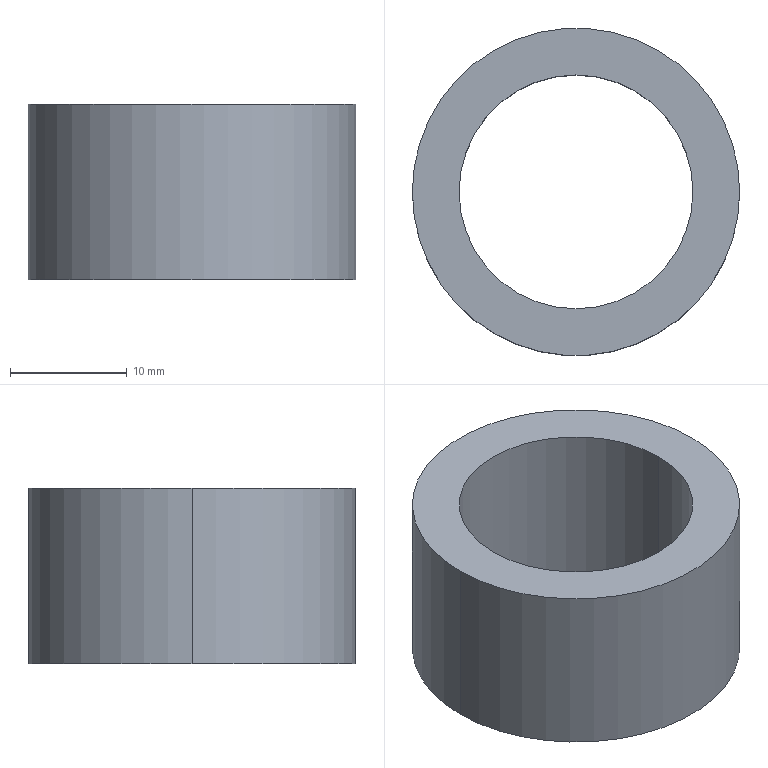Component | SolidWorks | GraphiteCopperSleeve1-1 | 1 solid | 6 faces | box 28 x 28 x 15 mm | volume 4524 mm3 | cylinder 4 | plane 2 | commonest cylinder face diameters 20 x2 28 x2
build123d program:
from build123d import *

# Parameters (mm, degrees)
SKETCH1_R           = 14
SKETCH1_R_2         = 10
BOSS_EXTRUDE1_DEPTH = 15


with BuildPart() as part:
    # Sketch1 → Boss-Extrude1 (new body)
    with BuildSketch(Plane.XY):
        Circle(SKETCH1_R)
        Circle(SKETCH1_R_2, mode=Mode.SUBTRACT)
    extrude(amount=BOSS_EXTRUDE1_DEPTH)


solid = part.part

# Placed as in the assembly
solid = solid.moved(Location((-372.766, -43.543, 915), (0, 0, 0)))
STEP:
#1=COLOUR_RGB('',0.7922,0.8196,0.9333);
#2=FILL_AREA_STYLE_COLOUR('',#1);
#3=FILL_AREA_STYLE('',(#2));
#4=SURFACE_STYLE_FILL_AREA(#3);
#5=SURFACE_SIDE_STYLE('',(#4));
#6=SURFACE_STYLE_USAGE(.BOTH.,#5);
#7=PRESENTATION_STYLE_ASSIGNMENT((#6));
#8=CARTESIAN_POINT('',(-15.07,-1.714,36.614));
#9=VERTEX_POINT('',#8);
#10=CARTESIAN_POINT('',(-14.282,-1.714,36.614));
#11=VERTEX_POINT('',#10);
#12=CARTESIAN_POINT('',(-14.676,-1.714,36.614));
#13=DIRECTION('',(0.,-0.,1.));
#14=DIRECTION('',(1.,0.,0.));
#15=AXIS2_PLACEMENT_3D('',#12,#13,#14);
#16=CIRCLE('',#15,0.3937);
#17=EDGE_CURVE('',#9,#11,#16,.T.);
#18=ORIENTED_EDGE('',*,*,#17,.T.);
#19=CARTESIAN_POINT('',(-14.282,-1.714,36.024));
#20=VERTEX_POINT('',#19);
#21=CARTESIAN_POINT('',(-14.282,-1.714,36.614));
#22=DIRECTION('',(-0.,0.,-1.));
#23=VECTOR('',#22,39.37);
#24=LINE('',#21,#23);
#25=EDGE_CURVE('',#11,#20,#24,.T.);
#26=ORIENTED_EDGE('',*,*,#25,.T.);
#27=CARTESIAN_POINT('',(-15.07,-1.714,36.024));
#28=VERTEX_POINT('',#27);
#29=CARTESIAN_POINT('',(-14.676,-1.714,36.024));
#30=DIRECTION('',(0.,-0.,1.));
#31=DIRECTION('',(1.,0.,0.));
#32=AXIS2_PLACEMENT_3D('',#29,#30,#31);
#33=CIRCLE('',#32,0.3937);
#34=EDGE_CURVE('',#28,#20,#33,.T.);
#35=ORIENTED_EDGE('',*,*,#34,.F.);
#36=CARTESIAN_POINT('',(-15.07,-1.714,36.614));
#37=DIRECTION('',(-0.,0.,-1.));
#38=VECTOR('',#37,39.37);
#39=LINE('',#36,#38);
#40=EDGE_CURVE('',#9,#28,#39,.T.);
#41=ORIENTED_EDGE('',*,*,#40,.F.);
#42=EDGE_LOOP('',(#18,#26,#35,#41));
#43=FACE_OUTER_BOUND('',#42,.T.);
#44=CARTESIAN_POINT('',(-14.676,-1.714,36.614));
#45=DIRECTION('',(-0.,0.,-1.));
#46=DIRECTION('',(-1.,-0.,0.));
#47=AXIS2_PLACEMENT_3D('',#44,#45,#46);
#48=CYLINDRICAL_SURFACE('',#47,0.3937);
#49=ADVANCED_FACE('',(#43),#48,.F.);
#50=CARTESIAN_POINT('',(-14.125,-1.714,36.614));
#51=VERTEX_POINT('',#50);
#52=CARTESIAN_POINT('',(-15.227,-1.714,36.614));
#53=VERTEX_POINT('',#52);
#54=CARTESIAN_POINT('',(-14.676,-1.714,36.614));
#55=DIRECTION('',(0.,-0.,1.));
#56=DIRECTION('',(1.,0.,0.));
#57=AXIS2_PLACEMENT_3D('',#54,#55,#56);
#58=CIRCLE('',#57,0.5512);
#59=EDGE_CURVE('',#51,#53,#58,.T.);
#60=ORIENTED_EDGE('',*,*,#59,.F.);
#61=CARTESIAN_POINT('',(-14.125,-1.714,36.024));
#62=VERTEX_POINT('',#61);
#63=CARTESIAN_POINT('',(-14.125,-1.714,36.614));
#64=DIRECTION('',(-0.,0.,-1.));
#65=VECTOR('',#64,39.37);
#66=LINE('',#63,#65);
#67=EDGE_CURVE('',#51,#62,#66,.T.);
#68=ORIENTED_EDGE('',*,*,#67,.T.);
#69=CARTESIAN_POINT('',(-15.227,-1.714,36.024));
#70=VERTEX_POINT('',#69);
#71=CARTESIAN_POINT('',(-14.676,-1.714,36.024));
#72=DIRECTION('',(0.,-0.,1.));
#73=DIRECTION('',(1.,0.,0.));
#74=AXIS2_PLACEMENT_3D('',#71,#72,#73);
#75=CIRCLE('',#74,0.5512);
#76=EDGE_CURVE('',#62,#70,#75,.T.);
#77=ORIENTED_EDGE('',*,*,#76,.T.);
#78=CARTESIAN_POINT('',(-15.227,-1.714,36.614));
#79=DIRECTION('',(-0.,0.,-1.));
#80=VECTOR('',#79,39.37);
#81=LINE('',#78,#80);
#82=EDGE_CURVE('',#53,#70,#81,.T.);
#83=ORIENTED_EDGE('',*,*,#82,.F.);
#84=EDGE_LOOP('',(#60,#68,#77,#83));
#85=FACE_OUTER_BOUND('',#84,.T.);
#86=CARTESIAN_POINT('',(-14.676,-1.714,36.614));
#87=DIRECTION('',(-0.,0.,-1.));
#88=DIRECTION('',(-1.,-0.,0.));
#89=AXIS2_PLACEMENT_3D('',#86,#87,#88);
#90=CYLINDRICAL_SURFACE('',#89,0.5512);
#91=ADVANCED_FACE('',(#85),#90,.T.);
#92=CARTESIAN_POINT('',(-14.676,-1.714,36.614));
#93=DIRECTION('',(0.,-0.,1.));
#94=DIRECTION('',(1.,0.,0.));
#95=AXIS2_PLACEMENT_3D('',#92,#93,#94);
#96=CIRCLE('',#95,0.5512);
#97=EDGE_CURVE('',#53,#51,#96,.T.);
#98=ORIENTED_EDGE('',*,*,#97,.T.);
#99=ORIENTED_EDGE('',*,*,#59,.T.);
#100=EDGE_LOOP('',(#98,#99));
#101=FACE_OUTER_BOUND('',#100,.T.);
#102=ORIENTED_EDGE('',*,*,#17,.F.);
#103=CARTESIAN_POINT('',(-14.676,-1.714,36.614));
#104=DIRECTION('',(0.,-0.,1.));
#105=DIRECTION('',(1.,0.,0.));
#106=AXIS2_PLACEMENT_3D('',#103,#104,#105);
#107=CIRCLE('',#106,0.3937);
#108=EDGE_CURVE('',#11,#9,#107,.T.);
#109=ORIENTED_EDGE('',*,*,#108,.F.);
#110=EDGE_LOOP('',(#102,#109));
#111=FACE_BOUND('',#110,.T.);
#112=CARTESIAN_POINT('',(-14.676,-1.714,36.614));
#113=DIRECTION('',(0.,-0.,1.));
#114=DIRECTION('',(1.,0.,-0.));
#115=AXIS2_PLACEMENT_3D('',#112,#113,#114);
#116=PLANE('',#115);
#117=ADVANCED_FACE('',(#101,#111),#116,.T.);
#118=CARTESIAN_POINT('',(-14.676,-1.714,36.024));
#119=DIRECTION('',(0.,-0.,1.));
#120=DIRECTION('',(1.,0.,0.));
#121=AXIS2_PLACEMENT_3D('',#118,#119,#120);
#122=CIRCLE('',#121,0.5512);
#123=EDGE_CURVE('',#70,#62,#122,.T.);
#124=ORIENTED_EDGE('',*,*,#123,.F.);
#125=ORIENTED_EDGE('',*,*,#76,.F.);
#126=EDGE_LOOP('',(#124,#125));
#127=FACE_OUTER_BOUND('',#126,.T.);
#128=ORIENTED_EDGE('',*,*,#34,.T.);
#129=CARTESIAN_POINT('',(-14.676,-1.714,36.024));
#130=DIRECTION('',(0.,-0.,1.));
#131=DIRECTION('',(1.,0.,0.));
#132=AXIS2_PLACEMENT_3D('',#129,#130,#131);
#133=CIRCLE('',#132,0.3937);
#134=EDGE_CURVE('',#20,#28,#133,.T.);
#135=ORIENTED_EDGE('',*,*,#134,.T.);
#136=EDGE_LOOP('',(#128,#135));
#137=FACE_BOUND('',#136,.T.);
#138=CARTESIAN_POINT('',(-14.676,-1.714,36.024));
#139=DIRECTION('',(0.,-0.,1.));
#140=DIRECTION('',(1.,0.,-0.));
#141=AXIS2_PLACEMENT_3D('',#138,#139,#140);
#142=PLANE('',#141);
#143=ADVANCED_FACE('',(#127,#137),#142,.F.);
#144=ORIENTED_EDGE('',*,*,#67,.F.);
#145=ORIENTED_EDGE('',*,*,#97,.F.);
#146=ORIENTED_EDGE('',*,*,#82,.T.);
#147=ORIENTED_EDGE('',*,*,#123,.T.);
#148=EDGE_LOOP('',(#144,#145,#146,#147));
#149=FACE_OUTER_BOUND('',#148,.T.);
#150=CARTESIAN_POINT('',(-14.676,-1.714,36.614));
#151=DIRECTION('',(-0.,0.,-1.));
#152=DIRECTION('',(-1.,-0.,0.));
#153=AXIS2_PLACEMENT_3D('',#150,#151,#152);
#154=CYLINDRICAL_SURFACE('',#153,0.5512);
#155=ADVANCED_FACE('',(#149),#154,.T.);
#156=ORIENTED_EDGE('',*,*,#25,.F.);
#157=ORIENTED_EDGE('',*,*,#108,.T.);
#158=ORIENTED_EDGE('',*,*,#40,.T.);
#159=ORIENTED_EDGE('',*,*,#134,.F.);
#160=EDGE_LOOP('',(#156,#157,#158,#159));
#161=FACE_OUTER_BOUND('',#160,.T.);
#162=CARTESIAN_POINT('',(-14.676,-1.714,36.614));
#163=DIRECTION('',(-0.,0.,-1.));
#164=DIRECTION('',(-1.,-0.,0.));
#165=AXIS2_PLACEMENT_3D('',#162,#163,#164);
#166=CYLINDRICAL_SURFACE('',#165,0.3937);
#167=ADVANCED_FACE('',(#161),#166,.F.);
#168=CLOSED_SHELL('',(#49,#91,#117,#143,#155,#167));
#169=MANIFOLD_SOLID_BREP('',#168);
#170=STYLED_ITEM('',(#7),#169);
#171=(LENGTH_UNIT()NAMED_UNIT(*)SI_UNIT($,.METRE.));
#172=LENGTH_MEASURE_WITH_UNIT(LENGTH_MEASURE(0.0254),#171);
#173=DIMENSIONAL_EXPONENTS(1.,0.,0.,0.,0.,0.,0.);
#174=(CONVERSION_BASED_UNIT('',#172)LENGTH_UNIT()NAMED_UNIT(#173));
#175=UNCERTAINTY_MEASURE_WITH_UNIT(LENGTH_MEASURE(0.00001),#174,'','');
#176=(NAMED_UNIT(*)PLANE_ANGLE_UNIT()SI_UNIT($,.RADIAN.));
#177=(NAMED_UNIT(*)SI_UNIT($,.STERADIAN.)SOLID_ANGLE_UNIT());
#178=(GEOMETRIC_REPRESENTATION_CONTEXT(3)GLOBAL_UNCERTAINTY_ASSIGNED_CONTEXT((#175))GLOBAL_UNIT_ASSIGNED_CONTEXT((#174,#176,#177))REPRESENTATION_CONTEXT('',''));
#179=MECHANICAL_DESIGN_GEOMETRIC_PRESENTATION_REPRESENTATION('',(#170),#178);
#180=CARTESIAN_POINT('',(0.,0.,0.));
#181=DIRECTION('',(0.,0.,1.));
#182=DIRECTION('',(1.,0.,0.));
#183=AXIS2_PLACEMENT_3D('',#180,#181,#182);
#184=(LENGTH_UNIT()NAMED_UNIT(*)SI_UNIT($,.METRE.));
#185=LENGTH_MEASURE_WITH_UNIT(LENGTH_MEASURE(0.0254),#184);
#186=DIMENSIONAL_EXPONENTS(1.,0.,0.,0.,0.,0.,0.);
#187=(CONVERSION_BASED_UNIT('',#185)LENGTH_UNIT()NAMED_UNIT(#186));
#188=UNCERTAINTY_MEASURE_WITH_UNIT(LENGTH_MEASURE(0.00001),#187,'','');
#189=(NAMED_UNIT(*)PLANE_ANGLE_UNIT()SI_UNIT($,.RADIAN.));
#190=(NAMED_UNIT(*)SI_UNIT($,.STERADIAN.)SOLID_ANGLE_UNIT());
#191=(GEOMETRIC_REPRESENTATION_CONTEXT(3)GLOBAL_UNCERTAINTY_ASSIGNED_CONTEXT((#188))GLOBAL_UNIT_ASSIGNED_CONTEXT((#187,#189,#190))REPRESENTATION_CONTEXT('',''));
#192=ADVANCED_BREP_SHAPE_REPRESENTATION('',(#169,#183),#191);
#193=PRESENTATION_LAYER_ASSIGNMENT('','',(#170));